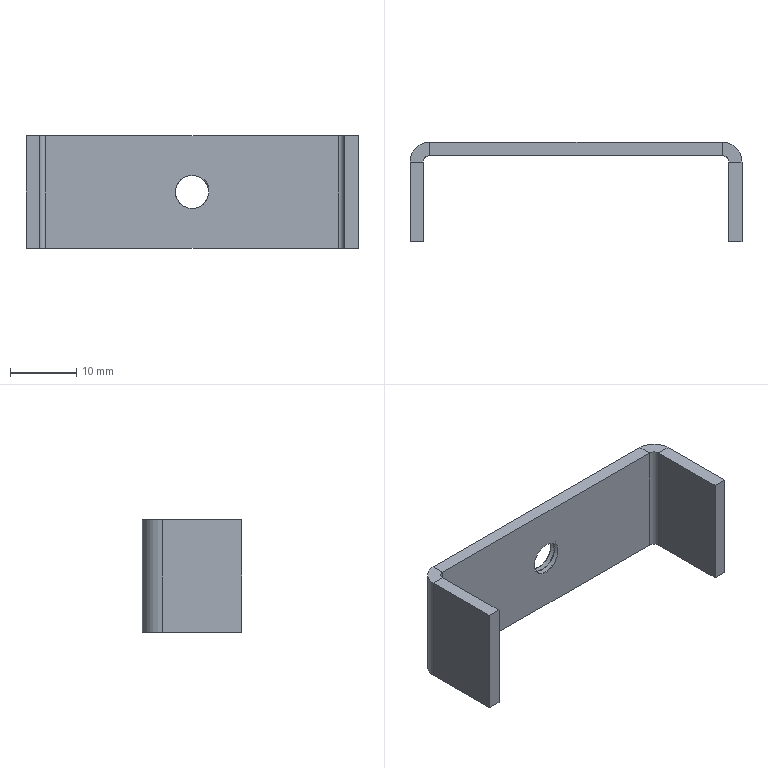Component | SolidWorks | CableClamp-1 | 1 solid | 31 faces | volume 2478 mm3 | plane 19 | cylinder 10 | spline 2 | commonest cylinder face diameters 5 x6 6 x2 2 x2